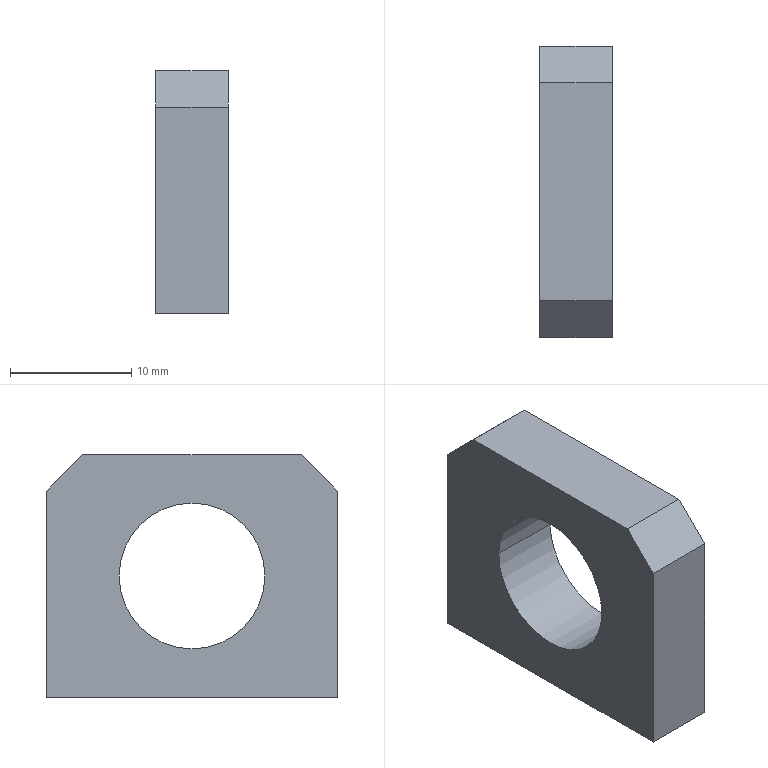Component | SolidWorks | JR-PL-JD-04CylinderFixingPlate-1 | 1 solid | 18 faces | box 6 x 24 x 20 mm | volume 2062 mm3 | plane 8 | cylinder 6 | cone 4 | commonest cylinder face diameters 2.5 x4 12 x2
build123d program:
from build123d import *

# Parameters (mm, degrees)
SKETCH1_W             = 24
SKETCH1_H             = 20
BOSS_EXTRUDE1_DEPTH   = 6
SKETCH2_R             = 6
CUT_EXTRUDE1_DEPTH    = 6
M3_TAPPED_HOLE1_D     = 2.5
M3_TAPPED_HOLE1_DEPTH = 8.5
M3_TAPPED_HOLE1_TIP   = 0.7511
CHAMFER1_SIZE         = 3


with BuildPart() as part:
    # Sketch1 → Boss-Extrude1 (new body)
    with BuildSketch(Plane.XY):
        with Locations((12, 10)):
            Rectangle(SKETCH1_W, SKETCH1_H)
    extrude(amount=BOSS_EXTRUDE1_DEPTH)

    # Sketch2 → Cut-Extrude1 (cut)
    with BuildSketch(Plane.XY.offset(6)):
        with Locations((12, 10)):
            Circle(SKETCH2_R)
    extrude(amount=-CUT_EXTRUDE1_DEPTH, mode=Mode.SUBTRACT)

    # M3 Tapped Hole1
    with Locations(Plane(origin=(0, 0, 0), x_dir=(-1, 0, 0), z_dir=(0, -1, 0))):
        with Locations((-19.5, -3), (-4.5, -3)):
            Hole(M3_TAPPED_HOLE1_D / 2, depth=M3_TAPPED_HOLE1_DEPTH)
            with Locations((0, 0, -(M3_TAPPED_HOLE1_DEPTH + M3_TAPPED_HOLE1_TIP / 2))):  # 118° drill point
                Cone(0, M3_TAPPED_HOLE1_D / 2, M3_TAPPED_HOLE1_TIP, mode=Mode.SUBTRACT)

    # Chamfer1
    chamfer1_edges = [part.edges().sort_by_distance(p)[0] for p in [
        (0, 20, 3),
        (24, 20, 3),
    ]]
    chamfer(chamfer1_edges, length=CHAMFER1_SIZE)


solid = part.part

# Placed as in the assembly
solid = solid.moved(Location((-13.325, 42.452, 62.77), (90, -90, 0)))
STEP:
#1=COLOUR_RGB('',0.7922,0.8196,0.9333);
#2=FILL_AREA_STYLE_COLOUR('',#1);
#3=FILL_AREA_STYLE('',(#2));
#4=SURFACE_STYLE_FILL_AREA(#3);
#5=SURFACE_SIDE_STYLE('',(#4));
#6=SURFACE_STYLE_USAGE(.BOTH.,#5);
#7=PRESENTATION_STYLE_ASSIGNMENT((#6));
#8=CARTESIAN_POINT('',(-0.6919,0.9036,2.806));
#9=VERTEX_POINT('',#8);
#10=CARTESIAN_POINT('',(-0.5935,0.9036,2.806));
#11=VERTEX_POINT('',#10);
#12=CARTESIAN_POINT('',(-0.6427,0.9036,2.806));
#13=DIRECTION('',(0.,0.,-1.));
#14=DIRECTION('',(1.,0.,0.));
#15=AXIS2_PLACEMENT_3D('',#12,#13,#14);
#16=CIRCLE('',#15,0.04921);
#17=EDGE_CURVE('',#9,#11,#16,.T.);
#18=ORIENTED_EDGE('',*,*,#17,.F.);
#19=CARTESIAN_POINT('',(-0.6919,0.9036,2.471));
#20=VERTEX_POINT('',#19);
#21=CARTESIAN_POINT('',(-0.6919,0.9036,2.471));
#22=DIRECTION('',(0.,0.,-1.));
#23=VECTOR('',#22,39.37);
#24=LINE('',#21,#23);
#25=EDGE_CURVE('',#9,#20,#24,.T.);
#26=ORIENTED_EDGE('',*,*,#25,.T.);
#27=CARTESIAN_POINT('',(-0.5935,0.9036,2.471));
#28=VERTEX_POINT('',#27);
#29=CARTESIAN_POINT('',(-0.6427,0.9036,2.471));
#30=DIRECTION('',(0.,0.,-1.));
#31=DIRECTION('',(1.,0.,0.));
#32=AXIS2_PLACEMENT_3D('',#29,#30,#31);
#33=CIRCLE('',#32,0.04921);
#34=EDGE_CURVE('',#20,#28,#33,.T.);
#35=ORIENTED_EDGE('',*,*,#34,.T.);
#36=CARTESIAN_POINT('',(-0.5935,0.9036,2.471));
#37=DIRECTION('',(0.,0.,-1.));
#38=VECTOR('',#37,39.37);
#39=LINE('',#36,#38);
#40=EDGE_CURVE('',#11,#28,#39,.T.);
#41=ORIENTED_EDGE('',*,*,#40,.F.);
#42=EDGE_LOOP('',(#18,#26,#35,#41));
#43=FACE_OUTER_BOUND('',#42,.T.);
#44=CARTESIAN_POINT('',(-0.6427,0.9036,2.471));
#45=DIRECTION('',(0.,0.,-1.));
#46=DIRECTION('',(1.,0.,0.));
#47=AXIS2_PLACEMENT_3D('',#44,#45,#46);
#48=CYLINDRICAL_SURFACE('',#47,0.04921);
#49=ADVANCED_FACE('',(#43),#48,.F.);
#50=CARTESIAN_POINT('',(-0.6427,0.9036,2.835));
#51=VERTEX_POINT('',#50);
#52=CARTESIAN_POINT('',(-0.5935,0.9036,2.806));
#53=DIRECTION('',(0.8572,0.,-0.515));
#54=VECTOR('',#53,39.37);
#55=LINE('',#52,#54);
#56=EDGE_CURVE('',#51,#11,#55,.T.);
#57=ORIENTED_EDGE('',*,*,#56,.F.);
#58=CARTESIAN_POINT('',(-0.6919,0.9036,2.806));
#59=DIRECTION('',(-0.8572,-0.,-0.515));
#60=VECTOR('',#59,39.37);
#61=LINE('',#58,#60);
#62=EDGE_CURVE('',#51,#9,#61,.T.);
#63=ORIENTED_EDGE('',*,*,#62,.T.);
#64=ORIENTED_EDGE('',*,*,#17,.T.);
#65=EDGE_LOOP('',(#57,#63,#64));
#66=FACE_OUTER_BOUND('',#65,.T.);
#67=CARTESIAN_POINT('',(-0.6427,0.9036,2.806));
#68=DIRECTION('',(0.,0.,-1.));
#69=DIRECTION('',(1.,0.,0.));
#70=AXIS2_PLACEMENT_3D('',#67,#68,#69);
#71=CONICAL_SURFACE('',#70,0.04921,1.03);
#72=ADVANCED_FACE('',(#66),#71,.F.);
#73=CARTESIAN_POINT('',(-0.6919,1.494,2.806));
#74=VERTEX_POINT('',#73);
#75=CARTESIAN_POINT('',(-0.5935,1.494,2.806));
#76=VERTEX_POINT('',#75);
#77=CARTESIAN_POINT('',(-0.6427,1.494,2.806));
#78=DIRECTION('',(0.,0.,-1.));
#79=DIRECTION('',(1.,0.,0.));
#80=AXIS2_PLACEMENT_3D('',#77,#78,#79);
#81=CIRCLE('',#80,0.04921);
#82=EDGE_CURVE('',#74,#76,#81,.T.);
#83=ORIENTED_EDGE('',*,*,#82,.F.);
#84=CARTESIAN_POINT('',(-0.6919,1.494,2.471));
#85=VERTEX_POINT('',#84);
#86=CARTESIAN_POINT('',(-0.6919,1.494,2.471));
#87=DIRECTION('',(0.,0.,-1.));
#88=VECTOR('',#87,39.37);
#89=LINE('',#86,#88);
#90=EDGE_CURVE('',#74,#85,#89,.T.);
#91=ORIENTED_EDGE('',*,*,#90,.T.);
#92=CARTESIAN_POINT('',(-0.5935,1.494,2.471));
#93=VERTEX_POINT('',#92);
#94=CARTESIAN_POINT('',(-0.6427,1.494,2.471));
#95=DIRECTION('',(0.,0.,-1.));
#96=DIRECTION('',(1.,0.,0.));
#97=AXIS2_PLACEMENT_3D('',#94,#95,#96);
#98=CIRCLE('',#97,0.04921);
#99=EDGE_CURVE('',#85,#93,#98,.T.);
#100=ORIENTED_EDGE('',*,*,#99,.T.);
#101=CARTESIAN_POINT('',(-0.5935,1.494,2.471));
#102=DIRECTION('',(0.,0.,-1.));
#103=VECTOR('',#102,39.37);
#104=LINE('',#101,#103);
#105=EDGE_CURVE('',#76,#93,#104,.T.);
#106=ORIENTED_EDGE('',*,*,#105,.F.);
#107=EDGE_LOOP('',(#83,#91,#100,#106));
#108=FACE_OUTER_BOUND('',#107,.T.);
#109=CARTESIAN_POINT('',(-0.6427,1.494,2.471));
#110=DIRECTION('',(0.,0.,-1.));
#111=DIRECTION('',(1.,0.,0.));
#112=AXIS2_PLACEMENT_3D('',#109,#110,#111);
#113=CYLINDRICAL_SURFACE('',#112,0.04921);
#114=ADVANCED_FACE('',(#108),#113,.F.);
#115=CARTESIAN_POINT('',(-0.6427,1.494,2.835));
#116=VERTEX_POINT('',#115);
#117=CARTESIAN_POINT('',(-0.5935,1.494,2.806));
#118=DIRECTION('',(0.8572,0.,-0.515));
#119=VECTOR('',#118,39.37);
#120=LINE('',#117,#119);
#121=EDGE_CURVE('',#116,#76,#120,.T.);
#122=ORIENTED_EDGE('',*,*,#121,.F.);
#123=CARTESIAN_POINT('',(-0.6919,1.494,2.806));
#124=DIRECTION('',(-0.8572,-0.,-0.515));
#125=VECTOR('',#124,39.37);
#126=LINE('',#123,#125);
#127=EDGE_CURVE('',#116,#74,#126,.T.);
#128=ORIENTED_EDGE('',*,*,#127,.T.);
#129=ORIENTED_EDGE('',*,*,#82,.T.);
#130=EDGE_LOOP('',(#122,#128,#129));
#131=FACE_OUTER_BOUND('',#130,.T.);
#132=CARTESIAN_POINT('',(-0.6427,1.494,2.806));
#133=DIRECTION('',(0.,0.,-1.));
#134=DIRECTION('',(1.,0.,0.));
#135=AXIS2_PLACEMENT_3D('',#132,#133,#134);
#136=CONICAL_SURFACE('',#135,0.04921,1.03);
#137=ADVANCED_FACE('',(#131),#136,.F.);
#138=CARTESIAN_POINT('',(-0.5246,1.435,2.865));
#139=VERTEX_POINT('',#138);
#140=CARTESIAN_POINT('',(-0.5246,0.9627,2.865));
#141=VERTEX_POINT('',#140);
#142=CARTESIAN_POINT('',(-0.5246,1.199,2.865));
#143=DIRECTION('',(-1.,0.,0.));
#144=DIRECTION('',(0.,-1.,0.));
#145=AXIS2_PLACEMENT_3D('',#142,#143,#144);
#146=CIRCLE('',#145,0.2362);
#147=EDGE_CURVE('',#139,#141,#146,.T.);
#148=ORIENTED_EDGE('',*,*,#147,.F.);
#149=CARTESIAN_POINT('',(-0.7608,1.435,2.865));
#150=VERTEX_POINT('',#149);
#151=CARTESIAN_POINT('',(-0.5246,1.435,2.865));
#152=DIRECTION('',(-1.,0.,0.));
#153=VECTOR('',#152,39.37);
#154=LINE('',#151,#153);
#155=EDGE_CURVE('',#139,#150,#154,.T.);
#156=ORIENTED_EDGE('',*,*,#155,.T.);
#157=CARTESIAN_POINT('',(-0.7608,0.9627,2.865));
#158=VERTEX_POINT('',#157);
#159=CARTESIAN_POINT('',(-0.7608,1.199,2.865));
#160=DIRECTION('',(-1.,0.,0.));
#161=DIRECTION('',(0.,-1.,0.));
#162=AXIS2_PLACEMENT_3D('',#159,#160,#161);
#163=CIRCLE('',#162,0.2362);
#164=EDGE_CURVE('',#150,#158,#163,.T.);
#165=ORIENTED_EDGE('',*,*,#164,.T.);
#166=CARTESIAN_POINT('',(-0.5246,0.9627,2.865));
#167=DIRECTION('',(-1.,0.,0.));
#168=VECTOR('',#167,39.37);
#169=LINE('',#166,#168);
#170=EDGE_CURVE('',#141,#158,#169,.T.);
#171=ORIENTED_EDGE('',*,*,#170,.F.);
#172=EDGE_LOOP('',(#148,#156,#165,#171));
#173=FACE_OUTER_BOUND('',#172,.T.);
#174=CARTESIAN_POINT('',(-0.5246,1.199,2.865));
#175=DIRECTION('',(-1.,0.,0.));
#176=DIRECTION('',(0.,-1.,0.));
#177=AXIS2_PLACEMENT_3D('',#174,#175,#176);
#178=CYLINDRICAL_SURFACE('',#177,0.2362);
#179=ADVANCED_FACE('',(#173),#178,.F.);
#180=CARTESIAN_POINT('',(-0.7608,1.671,3.141));
#181=VERTEX_POINT('',#180);
#182=CARTESIAN_POINT('',(-0.7608,1.671,2.471));
#183=VERTEX_POINT('',#182);
#184=CARTESIAN_POINT('',(-0.7608,1.671,2.471));
#185=DIRECTION('',(0.,0.,-1.));
#186=VECTOR('',#185,39.37);
#187=LINE('',#184,#186);
#188=EDGE_CURVE('',#181,#183,#187,.T.);
#189=ORIENTED_EDGE('',*,*,#188,.F.);
#190=CARTESIAN_POINT('',(-0.5246,1.671,3.141));
#191=VERTEX_POINT('',#190);
#192=CARTESIAN_POINT('',(-0.7608,1.671,3.141));
#193=DIRECTION('',(1.,0.,0.));
#194=VECTOR('',#193,39.37);
#195=LINE('',#192,#194);
#196=EDGE_CURVE('',#181,#191,#195,.T.);
#197=ORIENTED_EDGE('',*,*,#196,.T.);
#198=CARTESIAN_POINT('',(-0.5246,1.671,2.471));
#199=VERTEX_POINT('',#198);
#200=CARTESIAN_POINT('',(-0.5246,1.671,2.471));
#201=DIRECTION('',(0.,0.,-1.));
#202=VECTOR('',#201,39.37);
#203=LINE('',#200,#202);
#204=EDGE_CURVE('',#191,#199,#203,.T.);
#205=ORIENTED_EDGE('',*,*,#204,.T.);
#206=CARTESIAN_POINT('',(-0.7608,1.671,2.471));
#207=DIRECTION('',(1.,0.,0.));
#208=VECTOR('',#207,39.37);
#209=LINE('',#206,#208);
#210=EDGE_CURVE('',#183,#199,#209,.T.);
#211=ORIENTED_EDGE('',*,*,#210,.F.);
#212=EDGE_LOOP('',(#189,#197,#205,#211));
#213=FACE_OUTER_BOUND('',#212,.T.);
#214=CARTESIAN_POINT('',(-0.7608,1.671,2.471));
#215=DIRECTION('',(0.,-1.,0.));
#216=DIRECTION('',(1.,0.,0.));
#217=AXIS2_PLACEMENT_3D('',#214,#215,#216);
#218=PLANE('',#217);
#219=ADVANCED_FACE('',(#213),#218,.F.);
#220=CARTESIAN_POINT('',(-0.6427,0.9036,2.471));
#221=DIRECTION('',(0.,0.,-1.));
#222=DIRECTION('',(1.,0.,0.));
#223=AXIS2_PLACEMENT_3D('',#220,#221,#222);
#224=CIRCLE('',#223,0.04921);
#225=EDGE_CURVE('',#28,#20,#224,.T.);
#226=ORIENTED_EDGE('',*,*,#225,.F.);
#227=ORIENTED_EDGE('',*,*,#34,.F.);
#228=EDGE_LOOP('',(#226,#227));
#229=FACE_BOUND('',#228,.T.);
#230=CARTESIAN_POINT('',(-0.6427,1.494,2.471));
#231=DIRECTION('',(0.,0.,-1.));
#232=DIRECTION('',(1.,0.,0.));
#233=AXIS2_PLACEMENT_3D('',#230,#231,#232);
#234=CIRCLE('',#233,0.04921);
#235=EDGE_CURVE('',#93,#85,#234,.T.);
#236=ORIENTED_EDGE('',*,*,#235,.F.);
#237=ORIENTED_EDGE('',*,*,#99,.F.);
#238=EDGE_LOOP('',(#236,#237));
#239=FACE_BOUND('',#238,.T.);
#240=CARTESIAN_POINT('',(-0.5246,0.7265,2.471));
#241=VERTEX_POINT('',#240);
#242=CARTESIAN_POINT('',(-0.5246,1.671,2.471));
#243=DIRECTION('',(0.,-1.,0.));
#244=VECTOR('',#243,39.37);
#245=LINE('',#242,#244);
#246=EDGE_CURVE('',#199,#241,#245,.T.);
#247=ORIENTED_EDGE('',*,*,#246,.T.);
#248=CARTESIAN_POINT('',(-0.7608,0.7265,2.471));
#249=VERTEX_POINT('',#248);
#250=CARTESIAN_POINT('',(-0.7608,0.7265,2.471));
#251=DIRECTION('',(1.,0.,0.));
#252=VECTOR('',#251,39.37);
#253=LINE('',#250,#252);
#254=EDGE_CURVE('',#249,#241,#253,.T.);
#255=ORIENTED_EDGE('',*,*,#254,.F.);
#256=CARTESIAN_POINT('',(-0.7608,1.671,2.471));
#257=DIRECTION('',(0.,-1.,0.));
#258=VECTOR('',#257,39.37);
#259=LINE('',#256,#258);
#260=EDGE_CURVE('',#183,#249,#259,.T.);
#261=ORIENTED_EDGE('',*,*,#260,.F.);
#262=ORIENTED_EDGE('',*,*,#210,.T.);
#263=EDGE_LOOP('',(#247,#255,#261,#262));
#264=FACE_OUTER_BOUND('',#263,.T.);
#265=CARTESIAN_POINT('',(-0.7608,1.671,2.471));
#266=DIRECTION('',(0.,0.,1.));
#267=DIRECTION('',(-1.,0.,0.));
#268=AXIS2_PLACEMENT_3D('',#265,#266,#267);
#269=PLANE('',#268);
#270=ADVANCED_FACE('',(#229,#239,#264),#269,.F.);
#271=CARTESIAN_POINT('',(-0.5246,0.7265,3.141));
#272=VERTEX_POINT('',#271);
#273=CARTESIAN_POINT('',(-0.5246,0.7265,2.471));
#274=DIRECTION('',(0.,0.,1.));
#275=VECTOR('',#274,39.37);
#276=LINE('',#273,#275);
#277=EDGE_CURVE('',#241,#272,#276,.T.);
#278=ORIENTED_EDGE('',*,*,#277,.T.);
#279=CARTESIAN_POINT('',(-0.7608,0.7265,3.141));
#280=VERTEX_POINT('',#279);
#281=CARTESIAN_POINT('',(-0.7608,0.7265,3.141));
#282=DIRECTION('',(-1.,0.,0.));
#283=VECTOR('',#282,39.37);
#284=LINE('',#281,#283);
#285=EDGE_CURVE('',#272,#280,#284,.T.);
#286=ORIENTED_EDGE('',*,*,#285,.T.);
#287=CARTESIAN_POINT('',(-0.7608,0.7265,2.471));
#288=DIRECTION('',(0.,0.,1.));
#289=VECTOR('',#288,39.37);
#290=LINE('',#287,#289);
#291=EDGE_CURVE('',#249,#280,#290,.T.);
#292=ORIENTED_EDGE('',*,*,#291,.F.);
#293=ORIENTED_EDGE('',*,*,#254,.T.);
#294=EDGE_LOOP('',(#278,#286,#292,#293));
#295=FACE_OUTER_BOUND('',#294,.T.);
#296=CARTESIAN_POINT('',(-0.7608,0.7265,2.471));
#297=DIRECTION('',(0.,1.,0.));
#298=DIRECTION('',(-1.,0.,0.));
#299=AXIS2_PLACEMENT_3D('',#296,#297,#298);
#300=PLANE('',#299);
#301=ADVANCED_FACE('',(#295),#300,.F.);
#302=CARTESIAN_POINT('',(-0.5246,0.8446,3.259));
#303=VERTEX_POINT('',#302);
#304=CARTESIAN_POINT('',(-0.5246,1.553,3.259));
#305=VERTEX_POINT('',#304);
#306=CARTESIAN_POINT('',(-0.5246,1.671,3.259));
#307=DIRECTION('',(0.,1.,0.));
#308=VECTOR('',#307,39.37);
#309=LINE('',#306,#308);
#310=EDGE_CURVE('',#303,#305,#309,.T.);
#311=ORIENTED_EDGE('',*,*,#310,.T.);
#312=CARTESIAN_POINT('',(-0.7608,1.553,3.259));
#313=VERTEX_POINT('',#312);
#314=CARTESIAN_POINT('',(-0.7608,1.553,3.259));
#315=DIRECTION('',(-1.,0.,0.));
#316=VECTOR('',#315,39.37);
#317=LINE('',#314,#316);
#318=EDGE_CURVE('',#305,#313,#317,.T.);
#319=ORIENTED_EDGE('',*,*,#318,.T.);
#320=CARTESIAN_POINT('',(-0.7608,0.8446,3.259));
#321=VERTEX_POINT('',#320);
#322=CARTESIAN_POINT('',(-0.7608,1.671,3.259));
#323=DIRECTION('',(0.,1.,0.));
#324=VECTOR('',#323,39.37);
#325=LINE('',#322,#324);
#326=EDGE_CURVE('',#321,#313,#325,.T.);
#327=ORIENTED_EDGE('',*,*,#326,.F.);
#328=CARTESIAN_POINT('',(-0.7608,0.8446,3.259));
#329=DIRECTION('',(1.,0.,0.));
#330=VECTOR('',#329,39.37);
#331=LINE('',#328,#330);
#332=EDGE_CURVE('',#321,#303,#331,.T.);
#333=ORIENTED_EDGE('',*,*,#332,.T.);
#334=EDGE_LOOP('',(#311,#319,#327,#333));
#335=FACE_OUTER_BOUND('',#334,.T.);
#336=CARTESIAN_POINT('',(-0.7608,1.671,3.259));
#337=DIRECTION('',(0.,0.,-1.));
#338=DIRECTION('',(1.,0.,0.));
#339=AXIS2_PLACEMENT_3D('',#336,#337,#338);
#340=PLANE('',#339);
#341=ADVANCED_FACE('',(#335),#340,.F.);
#342=CARTESIAN_POINT('',(-0.7608,1.199,2.865));
#343=DIRECTION('',(-1.,0.,0.));
#344=DIRECTION('',(0.,-1.,0.));
#345=AXIS2_PLACEMENT_3D('',#342,#343,#344);
#346=CIRCLE('',#345,0.2362);
#347=EDGE_CURVE('',#158,#150,#346,.T.);
#348=ORIENTED_EDGE('',*,*,#347,.F.);
#349=ORIENTED_EDGE('',*,*,#164,.F.);
#350=EDGE_LOOP('',(#348,#349));
#351=FACE_BOUND('',#350,.T.);
#352=ORIENTED_EDGE('',*,*,#326,.T.);
#353=CARTESIAN_POINT('',(-0.7608,1.671,3.141));
#354=DIRECTION('',(0.,0.7071,-0.7071));
#355=VECTOR('',#354,39.37);
#356=LINE('',#353,#355);
#357=EDGE_CURVE('',#313,#181,#356,.T.);
#358=ORIENTED_EDGE('',*,*,#357,.T.);
#359=ORIENTED_EDGE('',*,*,#188,.T.);
#360=ORIENTED_EDGE('',*,*,#260,.T.);
#361=ORIENTED_EDGE('',*,*,#291,.T.);
#362=CARTESIAN_POINT('',(-0.7608,0.8446,3.259));
#363=DIRECTION('',(0.,0.7071,0.7071));
#364=VECTOR('',#363,39.37);
#365=LINE('',#362,#364);
#366=EDGE_CURVE('',#280,#321,#365,.T.);
#367=ORIENTED_EDGE('',*,*,#366,.T.);
#368=EDGE_LOOP('',(#352,#358,#359,#360,#361,#367));
#369=FACE_OUTER_BOUND('',#368,.T.);
#370=CARTESIAN_POINT('',(-0.7608,1.671,2.471));
#371=DIRECTION('',(1.,0.,0.));
#372=DIRECTION('',(0.,1.,0.));
#373=AXIS2_PLACEMENT_3D('',#370,#371,#372);
#374=PLANE('',#373);
#375=ADVANCED_FACE('',(#351,#369),#374,.F.);
#376=CARTESIAN_POINT('',(-0.5246,1.199,2.865));
#377=DIRECTION('',(-1.,0.,0.));
#378=DIRECTION('',(0.,-1.,0.));
#379=AXIS2_PLACEMENT_3D('',#376,#377,#378);
#380=CIRCLE('',#379,0.2362);
#381=EDGE_CURVE('',#141,#139,#380,.T.);
#382=ORIENTED_EDGE('',*,*,#381,.T.);
#383=ORIENTED_EDGE('',*,*,#147,.T.);
#384=EDGE_LOOP('',(#382,#383));
#385=FACE_BOUND('',#384,.T.);
#386=ORIENTED_EDGE('',*,*,#204,.F.);
#387=CARTESIAN_POINT('',(-0.5246,2.006,2.806));
#388=DIRECTION('',(0.,-0.7071,0.7071));
#389=VECTOR('',#388,39.37);
#390=LINE('',#387,#389);
#391=EDGE_CURVE('',#191,#305,#390,.T.);
#392=ORIENTED_EDGE('',*,*,#391,.T.);
#393=ORIENTED_EDGE('',*,*,#310,.F.);
#394=CARTESIAN_POINT('',(-0.5246,0.8643,3.278));
#395=DIRECTION('',(0.,-0.7071,-0.7071));
#396=VECTOR('',#395,39.37);
#397=LINE('',#394,#396);
#398=EDGE_CURVE('',#303,#272,#397,.T.);
#399=ORIENTED_EDGE('',*,*,#398,.T.);
#400=ORIENTED_EDGE('',*,*,#277,.F.);
#401=ORIENTED_EDGE('',*,*,#246,.F.);
#402=EDGE_LOOP('',(#386,#392,#393,#399,#400,#401));
#403=FACE_OUTER_BOUND('',#402,.T.);
#404=CARTESIAN_POINT('',(-0.5246,1.671,2.471));
#405=DIRECTION('',(1.,0.,0.));
#406=DIRECTION('',(0.,1.,0.));
#407=AXIS2_PLACEMENT_3D('',#404,#405,#406);
#408=PLANE('',#407);
#409=ADVANCED_FACE('',(#385,#403),#408,.T.);
#410=ORIENTED_EDGE('',*,*,#155,.F.);
#411=ORIENTED_EDGE('',*,*,#381,.F.);
#412=ORIENTED_EDGE('',*,*,#170,.T.);
#413=ORIENTED_EDGE('',*,*,#347,.T.);
#414=EDGE_LOOP('',(#410,#411,#412,#413));
#415=FACE_OUTER_BOUND('',#414,.T.);
#416=CARTESIAN_POINT('',(-0.5246,1.199,2.865));
#417=DIRECTION('',(-1.,0.,0.));
#418=DIRECTION('',(0.,-1.,0.));
#419=AXIS2_PLACEMENT_3D('',#416,#417,#418);
#420=CYLINDRICAL_SURFACE('',#419,0.2362);
#421=ADVANCED_FACE('',(#415),#420,.F.);
#422=ORIENTED_EDGE('',*,*,#127,.F.);
#423=ORIENTED_EDGE('',*,*,#121,.T.);
#424=CARTESIAN_POINT('',(-0.6427,1.494,2.806));
#425=DIRECTION('',(0.,0.,-1.));
#426=DIRECTION('',(1.,0.,0.));
#427=AXIS2_PLACEMENT_3D('',#424,#425,#426);
#428=CIRCLE('',#427,0.04921);
#429=EDGE_CURVE('',#76,#74,#428,.T.);
#430=ORIENTED_EDGE('',*,*,#429,.T.);
#431=EDGE_LOOP('',(#422,#423,#430));
#432=FACE_OUTER_BOUND('',#431,.T.);
#433=CARTESIAN_POINT('',(-0.6427,1.494,2.806));
#434=DIRECTION('',(0.,0.,-1.));
#435=DIRECTION('',(1.,0.,0.));
#436=AXIS2_PLACEMENT_3D('',#433,#434,#435);
#437=CONICAL_SURFACE('',#436,0.04921,1.03);
#438=ADVANCED_FACE('',(#432),#437,.F.);
#439=ORIENTED_EDGE('',*,*,#90,.F.);
#440=ORIENTED_EDGE('',*,*,#429,.F.);
#441=ORIENTED_EDGE('',*,*,#105,.T.);
#442=ORIENTED_EDGE('',*,*,#235,.T.);
#443=EDGE_LOOP('',(#439,#440,#441,#442));
#444=FACE_OUTER_BOUND('',#443,.T.);
#445=CARTESIAN_POINT('',(-0.6427,1.494,2.471));
#446=DIRECTION('',(0.,0.,-1.));
#447=DIRECTION('',(1.,0.,0.));
#448=AXIS2_PLACEMENT_3D('',#445,#446,#447);
#449=CYLINDRICAL_SURFACE('',#448,0.04921);
#450=ADVANCED_FACE('',(#444),#449,.F.);
#451=ORIENTED_EDGE('',*,*,#62,.F.);
#452=ORIENTED_EDGE('',*,*,#56,.T.);
#453=CARTESIAN_POINT('',(-0.6427,0.9036,2.806));
#454=DIRECTION('',(0.,0.,-1.));
#455=DIRECTION('',(1.,0.,0.));
#456=AXIS2_PLACEMENT_3D('',#453,#454,#455);
#457=CIRCLE('',#456,0.04921);
#458=EDGE_CURVE('',#11,#9,#457,.T.);
#459=ORIENTED_EDGE('',*,*,#458,.T.);
#460=EDGE_LOOP('',(#451,#452,#459));
#461=FACE_OUTER_BOUND('',#460,.T.);
#462=CARTESIAN_POINT('',(-0.6427,0.9036,2.806));
#463=DIRECTION('',(0.,0.,-1.));
#464=DIRECTION('',(1.,0.,0.));
#465=AXIS2_PLACEMENT_3D('',#462,#463,#464);
#466=CONICAL_SURFACE('',#465,0.04921,1.03);
#467=ADVANCED_FACE('',(#461),#466,.F.);
#468=ORIENTED_EDGE('',*,*,#25,.F.);
#469=ORIENTED_EDGE('',*,*,#458,.F.);
#470=ORIENTED_EDGE('',*,*,#40,.T.);
#471=ORIENTED_EDGE('',*,*,#225,.T.);
#472=EDGE_LOOP('',(#468,#469,#470,#471));
#473=FACE_OUTER_BOUND('',#472,.T.);
#474=CARTESIAN_POINT('',(-0.6427,0.9036,2.471));
#475=DIRECTION('',(0.,0.,-1.));
#476=DIRECTION('',(1.,0.,0.));
#477=AXIS2_PLACEMENT_3D('',#474,#475,#476);
#478=CYLINDRICAL_SURFACE('',#477,0.04921);
#479=ADVANCED_FACE('',(#473),#478,.F.);
#480=ORIENTED_EDGE('',*,*,#357,.F.);
#481=ORIENTED_EDGE('',*,*,#318,.F.);
#482=ORIENTED_EDGE('',*,*,#391,.F.);
#483=ORIENTED_EDGE('',*,*,#196,.F.);
#484=EDGE_LOOP('',(#480,#481,#482,#483));
#485=FACE_OUTER_BOUND('',#484,.T.);
#486=CARTESIAN_POINT('',(-0.7608,1.671,3.141));
#487=DIRECTION('',(0.,-0.7071,-0.7071));
#488=DIRECTION('',(1.,0.,0.));
#489=AXIS2_PLACEMENT_3D('',#486,#487,#488);
#490=PLANE('',#489);
#491=ADVANCED_FACE('',(#485),#490,.F.);
#492=ORIENTED_EDGE('',*,*,#366,.F.);
#493=ORIENTED_EDGE('',*,*,#285,.F.);
#494=ORIENTED_EDGE('',*,*,#398,.F.);
#495=ORIENTED_EDGE('',*,*,#332,.F.);
#496=EDGE_LOOP('',(#492,#493,#494,#495));
#497=FACE_OUTER_BOUND('',#496,.T.);
#498=CARTESIAN_POINT('',(-0.7608,0.8446,3.259));
#499=DIRECTION('',(0.,0.7071,-0.7071));
#500=DIRECTION('',(1.,0.,0.));
#501=AXIS2_PLACEMENT_3D('',#498,#499,#500);
#502=PLANE('',#501);
#503=ADVANCED_FACE('',(#497),#502,.F.);
#504=CLOSED_SHELL('',(#49,#72,#114,#137,#179,#219,#270,#301,#341,#375,#409,#421,#438,#450,#467,#479,#491,#503));
#505=MANIFOLD_SOLID_BREP('',#504);
#506=STYLED_ITEM('',(#7),#505);
#507=(LENGTH_UNIT()NAMED_UNIT(*)SI_UNIT($,.METRE.));
#508=LENGTH_MEASURE_WITH_UNIT(LENGTH_MEASURE(0.0254),#507);
#509=DIMENSIONAL_EXPONENTS(1.,0.,0.,0.,0.,0.,0.);
#510=(CONVERSION_BASED_UNIT('',#508)LENGTH_UNIT()NAMED_UNIT(#509));
#511=UNCERTAINTY_MEASURE_WITH_UNIT(LENGTH_MEASURE(0.00001),#510,'','');
#512=(NAMED_UNIT(*)PLANE_ANGLE_UNIT()SI_UNIT($,.RADIAN.));
#513=(NAMED_UNIT(*)SI_UNIT($,.STERADIAN.)SOLID_ANGLE_UNIT());
#514=(GEOMETRIC_REPRESENTATION_CONTEXT(3)GLOBAL_UNCERTAINTY_ASSIGNED_CONTEXT((#511))GLOBAL_UNIT_ASSIGNED_CONTEXT((#510,#512,#513))REPRESENTATION_CONTEXT('',''));
#515=MECHANICAL_DESIGN_GEOMETRIC_PRESENTATION_REPRESENTATION('',(#506),#514);
#516=CARTESIAN_POINT('',(0.,0.,0.));
#517=DIRECTION('',(0.,0.,1.));
#518=DIRECTION('',(1.,0.,0.));
#519=AXIS2_PLACEMENT_3D('',#516,#517,#518);
#520=(LENGTH_UNIT()NAMED_UNIT(*)SI_UNIT($,.METRE.));
#521=LENGTH_MEASURE_WITH_UNIT(LENGTH_MEASURE(0.0254),#520);
#522=DIMENSIONAL_EXPONENTS(1.,0.,0.,0.,0.,0.,0.);
#523=(CONVERSION_BASED_UNIT('',#521)LENGTH_UNIT()NAMED_UNIT(#522));
#524=UNCERTAINTY_MEASURE_WITH_UNIT(LENGTH_MEASURE(0.00001),#523,'','');
#525=(NAMED_UNIT(*)PLANE_ANGLE_UNIT()SI_UNIT($,.RADIAN.));
#526=(NAMED_UNIT(*)SI_UNIT($,.STERADIAN.)SOLID_ANGLE_UNIT());
#527=(GEOMETRIC_REPRESENTATION_CONTEXT(3)GLOBAL_UNCERTAINTY_ASSIGNED_CONTEXT((#524))GLOBAL_UNIT_ASSIGNED_CONTEXT((#523,#525,#526))REPRESENTATION_CONTEXT('',''));
#528=ADVANCED_BREP_SHAPE_REPRESENTATION('',(#505,#519),#527);
#529=PRESENTATION_LAYER_ASSIGNMENT('','',(#506));